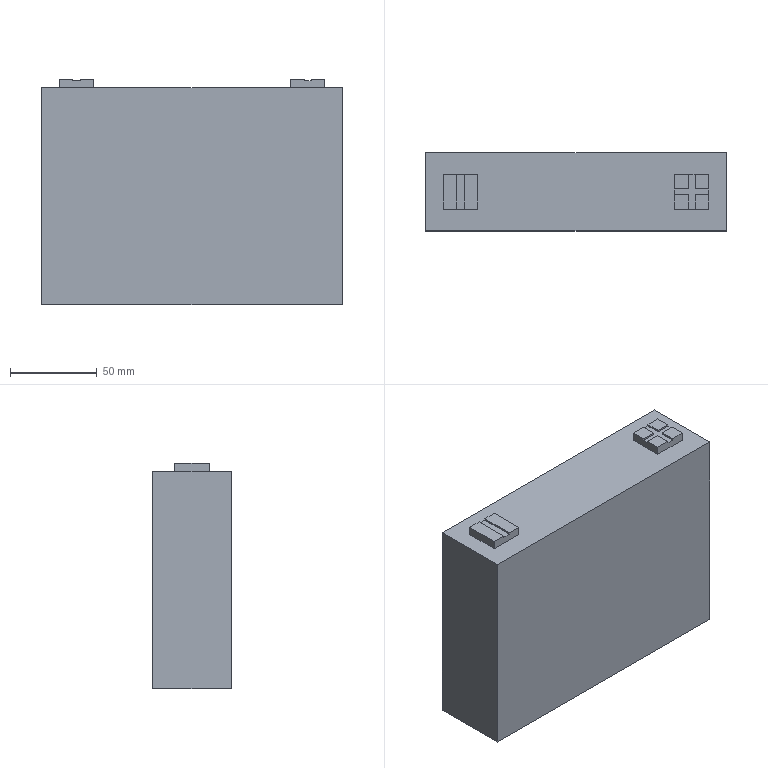Component | SolidWorks | AD12-SquareCell.SDPRT-15 | 1 solid | 32 faces | box 173 x 45 x 130 mm | volume 976901 mm3 | plane 32 | material 6061-T6 (SS)
build123d program:
from build123d import *

# Parameters (mm, degrees)
SKETCH1_W           = 173
SKETCH1_H           = 45
BOSS_EXTRUDE1_DEPTH = 125
SKETCH2_W           = 20
SKETCH2_H           = 20
BOSS_EXTRUDE2_DEPTH = 5
SKETCH3_W           = 4.63
SKETCH3_H           = 20
CUT_EXTRUDE1_DEPTH  = 1


with BuildPart() as part:
    # Sketch1 → Boss-Extrude1 (new body)
    with BuildSketch(Plane.XY):
        with Locations((86.5, 22.5)):
            Rectangle(SKETCH1_W, SKETCH1_H)
    extrude(amount=BOSS_EXTRUDE1_DEPTH)

    # Sketch2 → Boss-Extrude2 (add)
    with BuildSketch(Plane.XY.offset(125)):
        with Locations((153, 22.5)):
            Rectangle(SKETCH2_W, SKETCH2_H)
        with Locations((20, 22.5)):
            Rectangle(SKETCH2_W, SKETCH2_H)
    extrude(amount=BOSS_EXTRUDE2_DEPTH)

    # Sketch3 → Cut-Extrude1 (cut)
    with BuildSketch(Plane.XY.offset(130)):
        Polygon((143, 24.199), (151.25, 24.199), (151.25, 32.5), (155.042, 32.5), (155.042, 24.199), (163, 24.199), (163, 20.751), (155.042, 20.751), (155.042, 12.5), (151.25, 12.5), (151.25, 20.751), (143, 20.751), align=None)
        with Locations((19.957, 22.5)):
            Rectangle(SKETCH3_W, SKETCH3_H)
    extrude(amount=-CUT_EXTRUDE1_DEPTH, mode=Mode.SUBTRACT)


solid = part.part

# Placed as in the assembly
solid = solid.moved(Location((-374.414, -123.961, 199.12), (0, 0, 0)))
STEP:
#1=COLOUR_RGB('',0.7922,0.8196,0.9333);
#2=FILL_AREA_STYLE_COLOUR('',#1);
#3=FILL_AREA_STYLE('',(#2));
#4=SURFACE_STYLE_FILL_AREA(#3);
#5=SURFACE_SIDE_STYLE('',(#4));
#6=SURFACE_STYLE_USAGE(.BOTH.,#5);
#7=PRESENTATION_STYLE_ASSIGNMENT((#6));
#8=CARTESIAN_POINT('',(-14.046,-3.601,12.957));
#9=VERTEX_POINT('',#8);
#10=CARTESIAN_POINT('',(-14.046,-4.388,12.957));
#11=VERTEX_POINT('',#10);
#12=CARTESIAN_POINT('',(-14.046,-3.601,12.957));
#13=DIRECTION('',(0.,-1.,0.));
#14=VECTOR('',#13,39.37);
#15=LINE('',#12,#14);
#16=EDGE_CURVE('',#9,#11,#15,.T.);
#17=ORIENTED_EDGE('',*,*,#16,.F.);
#18=CARTESIAN_POINT('',(-14.347,-3.601,12.957));
#19=VERTEX_POINT('',#18);
#20=CARTESIAN_POINT('',(-14.347,-3.601,12.957));
#21=DIRECTION('',(-1.,0.,0.));
#22=VECTOR('',#21,39.37);
#23=LINE('',#20,#22);
#24=EDGE_CURVE('',#9,#19,#23,.T.);
#25=ORIENTED_EDGE('',*,*,#24,.T.);
#26=CARTESIAN_POINT('',(-14.347,-4.388,12.957));
#27=VERTEX_POINT('',#26);
#28=CARTESIAN_POINT('',(-14.347,-3.601,12.957));
#29=DIRECTION('',(0.,-1.,0.));
#30=VECTOR('',#29,39.37);
#31=LINE('',#28,#30);
#32=EDGE_CURVE('',#19,#27,#31,.T.);
#33=ORIENTED_EDGE('',*,*,#32,.T.);
#34=CARTESIAN_POINT('',(-14.347,-4.388,12.957));
#35=DIRECTION('',(1.,0.,0.));
#36=VECTOR('',#35,39.37);
#37=LINE('',#34,#36);
#38=EDGE_CURVE('',#27,#11,#37,.T.);
#39=ORIENTED_EDGE('',*,*,#38,.T.);
#40=EDGE_LOOP('',(#17,#25,#33,#39));
#41=FACE_OUTER_BOUND('',#40,.T.);
#42=CARTESIAN_POINT('',(-14.741,-4.88,12.957));
#43=DIRECTION('',(0.,0.,1.));
#44=DIRECTION('',(1.,0.,0.));
#45=AXIS2_PLACEMENT_3D('',#42,#43,#44);
#46=PLANE('',#45);
#47=ADVANCED_FACE('',(#41),#46,.T.);
#48=CARTESIAN_POINT('',(-8.786,-3.928,12.957));
#49=VERTEX_POINT('',#48);
#50=CARTESIAN_POINT('',(-9.111,-3.928,12.957));
#51=VERTEX_POINT('',#50);
#52=CARTESIAN_POINT('',(-9.111,-3.928,12.957));
#53=DIRECTION('',(-1.,0.,0.));
#54=VECTOR('',#53,39.37);
#55=LINE('',#52,#54);
#56=EDGE_CURVE('',#49,#51,#55,.T.);
#57=ORIENTED_EDGE('',*,*,#56,.F.);
#58=CARTESIAN_POINT('',(-8.786,-3.601,12.957));
#59=VERTEX_POINT('',#58);
#60=CARTESIAN_POINT('',(-8.786,-3.601,12.957));
#61=DIRECTION('',(0.,-1.,0.));
#62=VECTOR('',#61,39.37);
#63=LINE('',#60,#62);
#64=EDGE_CURVE('',#59,#49,#63,.T.);
#65=ORIENTED_EDGE('',*,*,#64,.F.);
#66=CARTESIAN_POINT('',(-9.111,-3.601,12.957));
#67=VERTEX_POINT('',#66);
#68=CARTESIAN_POINT('',(-9.111,-3.601,12.957));
#69=DIRECTION('',(-1.,0.,0.));
#70=VECTOR('',#69,39.37);
#71=LINE('',#68,#70);
#72=EDGE_CURVE('',#59,#67,#71,.T.);
#73=ORIENTED_EDGE('',*,*,#72,.T.);
#74=CARTESIAN_POINT('',(-9.111,-3.601,12.957));
#75=DIRECTION('',(0.,-1.,0.));
#76=VECTOR('',#75,39.37);
#77=LINE('',#74,#76);
#78=EDGE_CURVE('',#67,#51,#77,.T.);
#79=ORIENTED_EDGE('',*,*,#78,.T.);
#80=EDGE_LOOP('',(#57,#65,#73,#79));
#81=FACE_OUTER_BOUND('',#80,.T.);
#82=CARTESIAN_POINT('',(-14.741,-4.88,12.957));
#83=DIRECTION('',(0.,0.,1.));
#84=DIRECTION('',(1.,0.,0.));
#85=AXIS2_PLACEMENT_3D('',#82,#83,#84);
#86=PLANE('',#85);
#87=ADVANCED_FACE('',(#81),#86,.T.);
#88=CARTESIAN_POINT('',(-8.637,-3.928,12.957));
#89=VERTEX_POINT('',#88);
#90=CARTESIAN_POINT('',(-8.637,-3.601,12.957));
#91=VERTEX_POINT('',#90);
#92=CARTESIAN_POINT('',(-8.637,-3.601,12.957));
#93=DIRECTION('',(0.,1.,0.));
#94=VECTOR('',#93,39.37);
#95=LINE('',#92,#94);
#96=EDGE_CURVE('',#89,#91,#95,.T.);
#97=ORIENTED_EDGE('',*,*,#96,.F.);
#98=CARTESIAN_POINT('',(-8.323,-3.928,12.957));
#99=VERTEX_POINT('',#98);
#100=CARTESIAN_POINT('',(-8.637,-3.928,12.957));
#101=DIRECTION('',(-1.,0.,0.));
#102=VECTOR('',#101,39.37);
#103=LINE('',#100,#102);
#104=EDGE_CURVE('',#99,#89,#103,.T.);
#105=ORIENTED_EDGE('',*,*,#104,.F.);
#106=CARTESIAN_POINT('',(-8.323,-3.601,12.957));
#107=VERTEX_POINT('',#106);
#108=CARTESIAN_POINT('',(-8.323,-3.601,12.957));
#109=DIRECTION('',(0.,1.,0.));
#110=VECTOR('',#109,39.37);
#111=LINE('',#108,#110);
#112=EDGE_CURVE('',#99,#107,#111,.T.);
#113=ORIENTED_EDGE('',*,*,#112,.T.);
#114=CARTESIAN_POINT('',(-9.111,-3.601,12.957));
#115=DIRECTION('',(-1.,0.,0.));
#116=VECTOR('',#115,39.37);
#117=LINE('',#114,#116);
#118=EDGE_CURVE('',#107,#91,#117,.T.);
#119=ORIENTED_EDGE('',*,*,#118,.T.);
#120=EDGE_LOOP('',(#97,#105,#113,#119));
#121=FACE_OUTER_BOUND('',#120,.T.);
#122=CARTESIAN_POINT('',(-14.741,-4.88,12.957));
#123=DIRECTION('',(0.,0.,1.));
#124=DIRECTION('',(1.,0.,0.));
#125=AXIS2_PLACEMENT_3D('',#122,#123,#124);
#126=PLANE('',#125);
#127=ADVANCED_FACE('',(#121),#126,.T.);
#128=CARTESIAN_POINT('',(-8.637,-4.063,12.957));
#129=VERTEX_POINT('',#128);
#130=CARTESIAN_POINT('',(-8.323,-4.063,12.957));
#131=VERTEX_POINT('',#130);
#132=CARTESIAN_POINT('',(-8.637,-4.063,12.957));
#133=DIRECTION('',(1.,0.,0.));
#134=VECTOR('',#133,39.37);
#135=LINE('',#132,#134);
#136=EDGE_CURVE('',#129,#131,#135,.T.);
#137=ORIENTED_EDGE('',*,*,#136,.F.);
#138=CARTESIAN_POINT('',(-8.637,-4.388,12.957));
#139=VERTEX_POINT('',#138);
#140=CARTESIAN_POINT('',(-8.637,-4.063,12.957));
#141=DIRECTION('',(0.,1.,0.));
#142=VECTOR('',#141,39.37);
#143=LINE('',#140,#142);
#144=EDGE_CURVE('',#139,#129,#143,.T.);
#145=ORIENTED_EDGE('',*,*,#144,.F.);
#146=CARTESIAN_POINT('',(-8.323,-4.388,12.957));
#147=VERTEX_POINT('',#146);
#148=CARTESIAN_POINT('',(-9.111,-4.388,12.957));
#149=DIRECTION('',(1.,0.,0.));
#150=VECTOR('',#149,39.37);
#151=LINE('',#148,#150);
#152=EDGE_CURVE('',#139,#147,#151,.T.);
#153=ORIENTED_EDGE('',*,*,#152,.T.);
#154=CARTESIAN_POINT('',(-8.323,-3.601,12.957));
#155=DIRECTION('',(0.,1.,0.));
#156=VECTOR('',#155,39.37);
#157=LINE('',#154,#156);
#158=EDGE_CURVE('',#147,#131,#157,.T.);
#159=ORIENTED_EDGE('',*,*,#158,.T.);
#160=EDGE_LOOP('',(#137,#145,#153,#159));
#161=FACE_OUTER_BOUND('',#160,.T.);
#162=CARTESIAN_POINT('',(-14.741,-4.88,12.957));
#163=DIRECTION('',(0.,0.,1.));
#164=DIRECTION('',(1.,0.,0.));
#165=AXIS2_PLACEMENT_3D('',#162,#163,#164);
#166=PLANE('',#165);
#167=ADVANCED_FACE('',(#161),#166,.T.);
#168=CARTESIAN_POINT('',(-9.111,-3.601,12.761));
#169=VERTEX_POINT('',#168);
#170=CARTESIAN_POINT('',(-9.111,-4.388,12.761));
#171=VERTEX_POINT('',#170);
#172=CARTESIAN_POINT('',(-9.111,-3.601,12.761));
#173=DIRECTION('',(0.,-1.,0.));
#174=VECTOR('',#173,39.37);
#175=LINE('',#172,#174);
#176=EDGE_CURVE('',#169,#171,#175,.T.);
#177=ORIENTED_EDGE('',*,*,#176,.F.);
#178=CARTESIAN_POINT('',(-8.323,-3.601,12.761));
#179=VERTEX_POINT('',#178);
#180=CARTESIAN_POINT('',(-9.111,-3.601,12.761));
#181=DIRECTION('',(-1.,0.,0.));
#182=VECTOR('',#181,39.37);
#183=LINE('',#180,#182);
#184=EDGE_CURVE('',#179,#169,#183,.T.);
#185=ORIENTED_EDGE('',*,*,#184,.F.);
#186=CARTESIAN_POINT('',(-8.323,-4.388,12.761));
#187=VERTEX_POINT('',#186);
#188=CARTESIAN_POINT('',(-8.323,-3.601,12.761));
#189=DIRECTION('',(0.,1.,0.));
#190=VECTOR('',#189,39.37);
#191=LINE('',#188,#190);
#192=EDGE_CURVE('',#187,#179,#191,.T.);
#193=ORIENTED_EDGE('',*,*,#192,.F.);
#194=CARTESIAN_POINT('',(-9.111,-4.388,12.761));
#195=DIRECTION('',(1.,0.,0.));
#196=VECTOR('',#195,39.37);
#197=LINE('',#194,#196);
#198=EDGE_CURVE('',#171,#187,#197,.T.);
#199=ORIENTED_EDGE('',*,*,#198,.F.);
#200=EDGE_LOOP('',(#177,#185,#193,#199));
#201=FACE_BOUND('',#200,.T.);
#202=CARTESIAN_POINT('',(-14.741,-3.109,12.761));
#203=VERTEX_POINT('',#202);
#204=CARTESIAN_POINT('',(-14.741,-4.88,12.761));
#205=VERTEX_POINT('',#204);
#206=CARTESIAN_POINT('',(-14.741,-4.88,12.761));
#207=DIRECTION('',(-0.,-1.,0.));
#208=VECTOR('',#207,39.37);
#209=LINE('',#206,#208);
#210=EDGE_CURVE('',#203,#205,#209,.T.);
#211=ORIENTED_EDGE('',*,*,#210,.T.);
#212=CARTESIAN_POINT('',(-7.93,-4.88,12.761));
#213=VERTEX_POINT('',#212);
#214=CARTESIAN_POINT('',(-14.741,-4.88,12.761));
#215=DIRECTION('',(1.,0.,0.));
#216=VECTOR('',#215,39.37);
#217=LINE('',#214,#216);
#218=EDGE_CURVE('',#205,#213,#217,.T.);
#219=ORIENTED_EDGE('',*,*,#218,.T.);
#220=CARTESIAN_POINT('',(-7.93,-3.109,12.761));
#221=VERTEX_POINT('',#220);
#222=CARTESIAN_POINT('',(-7.93,-4.88,12.761));
#223=DIRECTION('',(0.,1.,0.));
#224=VECTOR('',#223,39.37);
#225=LINE('',#222,#224);
#226=EDGE_CURVE('',#213,#221,#225,.T.);
#227=ORIENTED_EDGE('',*,*,#226,.T.);
#228=CARTESIAN_POINT('',(-14.741,-3.109,12.761));
#229=DIRECTION('',(-1.,0.,0.));
#230=VECTOR('',#229,39.37);
#231=LINE('',#228,#230);
#232=EDGE_CURVE('',#221,#203,#231,.T.);
#233=ORIENTED_EDGE('',*,*,#232,.T.);
#234=EDGE_LOOP('',(#211,#219,#227,#233));
#235=FACE_OUTER_BOUND('',#234,.T.);
#236=CARTESIAN_POINT('',(-14.347,-3.601,12.761));
#237=VERTEX_POINT('',#236);
#238=CARTESIAN_POINT('',(-14.347,-4.388,12.761));
#239=VERTEX_POINT('',#238);
#240=CARTESIAN_POINT('',(-14.347,-3.601,12.761));
#241=DIRECTION('',(0.,-1.,0.));
#242=VECTOR('',#241,39.37);
#243=LINE('',#240,#242);
#244=EDGE_CURVE('',#237,#239,#243,.T.);
#245=ORIENTED_EDGE('',*,*,#244,.F.);
#246=CARTESIAN_POINT('',(-13.56,-3.601,12.761));
#247=VERTEX_POINT('',#246);
#248=CARTESIAN_POINT('',(-14.347,-3.601,12.761));
#249=DIRECTION('',(-1.,0.,0.));
#250=VECTOR('',#249,39.37);
#251=LINE('',#248,#250);
#252=EDGE_CURVE('',#247,#237,#251,.T.);
#253=ORIENTED_EDGE('',*,*,#252,.F.);
#254=CARTESIAN_POINT('',(-13.56,-4.388,12.761));
#255=VERTEX_POINT('',#254);
#256=CARTESIAN_POINT('',(-13.56,-3.601,12.761));
#257=DIRECTION('',(-0.,1.,0.));
#258=VECTOR('',#257,39.37);
#259=LINE('',#256,#258);
#260=EDGE_CURVE('',#255,#247,#259,.T.);
#261=ORIENTED_EDGE('',*,*,#260,.F.);
#262=CARTESIAN_POINT('',(-14.347,-4.388,12.761));
#263=DIRECTION('',(1.,0.,0.));
#264=VECTOR('',#263,39.37);
#265=LINE('',#262,#264);
#266=EDGE_CURVE('',#239,#255,#265,.T.);
#267=ORIENTED_EDGE('',*,*,#266,.F.);
#268=EDGE_LOOP('',(#245,#253,#261,#267));
#269=FACE_BOUND('',#268,.T.);
#270=CARTESIAN_POINT('',(-14.741,-4.88,12.761));
#271=DIRECTION('',(0.,0.,-1.));
#272=DIRECTION('',(-1.,0.,0.));
#273=AXIS2_PLACEMENT_3D('',#270,#271,#272);
#274=PLANE('',#273);
#275=ADVANCED_FACE('',(#201,#235,#269),#274,.F.);
#276=CARTESIAN_POINT('',(-14.741,-3.109,7.839));
#277=VERTEX_POINT('',#276);
#278=CARTESIAN_POINT('',(-14.741,-4.88,7.839));
#279=VERTEX_POINT('',#278);
#280=CARTESIAN_POINT('',(-14.741,-4.88,7.839));
#281=DIRECTION('',(-0.,-1.,0.));
#282=VECTOR('',#281,39.37);
#283=LINE('',#280,#282);
#284=EDGE_CURVE('',#277,#279,#283,.T.);
#285=ORIENTED_EDGE('',*,*,#284,.T.);
#286=CARTESIAN_POINT('',(-14.741,-4.88,12.761));
#287=DIRECTION('',(0.,0.,-1.));
#288=VECTOR('',#287,39.37);
#289=LINE('',#286,#288);
#290=EDGE_CURVE('',#205,#279,#289,.T.);
#291=ORIENTED_EDGE('',*,*,#290,.F.);
#292=ORIENTED_EDGE('',*,*,#210,.F.);
#293=CARTESIAN_POINT('',(-14.741,-3.109,12.761));
#294=DIRECTION('',(0.,0.,-1.));
#295=VECTOR('',#294,39.37);
#296=LINE('',#293,#295);
#297=EDGE_CURVE('',#203,#277,#296,.T.);
#298=ORIENTED_EDGE('',*,*,#297,.T.);
#299=EDGE_LOOP('',(#285,#291,#292,#298));
#300=FACE_OUTER_BOUND('',#299,.T.);
#301=CARTESIAN_POINT('',(-14.741,-4.88,12.761));
#302=DIRECTION('',(1.,-0.,0.));
#303=DIRECTION('',(0.,1.,0.));
#304=AXIS2_PLACEMENT_3D('',#301,#302,#303);
#305=PLANE('',#304);
#306=ADVANCED_FACE('',(#300),#305,.F.);
#307=CARTESIAN_POINT('',(-7.93,-4.88,7.839));
#308=VERTEX_POINT('',#307);
#309=CARTESIAN_POINT('',(-14.741,-4.88,7.839));
#310=DIRECTION('',(1.,0.,0.));
#311=VECTOR('',#310,39.37);
#312=LINE('',#309,#311);
#313=EDGE_CURVE('',#279,#308,#312,.T.);
#314=ORIENTED_EDGE('',*,*,#313,.T.);
#315=CARTESIAN_POINT('',(-7.93,-4.88,12.761));
#316=DIRECTION('',(0.,0.,-1.));
#317=VECTOR('',#316,39.37);
#318=LINE('',#315,#317);
#319=EDGE_CURVE('',#213,#308,#318,.T.);
#320=ORIENTED_EDGE('',*,*,#319,.F.);
#321=ORIENTED_EDGE('',*,*,#218,.F.);
#322=ORIENTED_EDGE('',*,*,#290,.T.);
#323=EDGE_LOOP('',(#314,#320,#321,#322));
#324=FACE_OUTER_BOUND('',#323,.T.);
#325=CARTESIAN_POINT('',(-14.741,-4.88,12.761));
#326=DIRECTION('',(0.,1.,0.));
#327=DIRECTION('',(0.,0.,1.));
#328=AXIS2_PLACEMENT_3D('',#325,#326,#327);
#329=PLANE('',#328);
#330=ADVANCED_FACE('',(#324),#329,.F.);
#331=CARTESIAN_POINT('',(-7.93,-3.109,7.839));
#332=VERTEX_POINT('',#331);
#333=CARTESIAN_POINT('',(-7.93,-4.88,7.839));
#334=DIRECTION('',(0.,1.,0.));
#335=VECTOR('',#334,39.37);
#336=LINE('',#333,#335);
#337=EDGE_CURVE('',#308,#332,#336,.T.);
#338=ORIENTED_EDGE('',*,*,#337,.T.);
#339=CARTESIAN_POINT('',(-7.93,-3.109,12.761));
#340=DIRECTION('',(0.,0.,-1.));
#341=VECTOR('',#340,39.37);
#342=LINE('',#339,#341);
#343=EDGE_CURVE('',#221,#332,#342,.T.);
#344=ORIENTED_EDGE('',*,*,#343,.F.);
#345=ORIENTED_EDGE('',*,*,#226,.F.);
#346=ORIENTED_EDGE('',*,*,#319,.T.);
#347=EDGE_LOOP('',(#338,#344,#345,#346));
#348=FACE_OUTER_BOUND('',#347,.T.);
#349=CARTESIAN_POINT('',(-7.93,-4.88,12.761));
#350=DIRECTION('',(-1.,0.,0.));
#351=DIRECTION('',(-0.,-1.,0.));
#352=AXIS2_PLACEMENT_3D('',#349,#350,#351);
#353=PLANE('',#352);
#354=ADVANCED_FACE('',(#348),#353,.F.);
#355=CARTESIAN_POINT('',(-14.741,-3.109,7.839));
#356=DIRECTION('',(-1.,0.,0.));
#357=VECTOR('',#356,39.37);
#358=LINE('',#355,#357);
#359=EDGE_CURVE('',#332,#277,#358,.T.);
#360=ORIENTED_EDGE('',*,*,#359,.T.);
#361=ORIENTED_EDGE('',*,*,#297,.F.);
#362=ORIENTED_EDGE('',*,*,#232,.F.);
#363=ORIENTED_EDGE('',*,*,#343,.T.);
#364=EDGE_LOOP('',(#360,#361,#362,#363));
#365=FACE_OUTER_BOUND('',#364,.T.);
#366=CARTESIAN_POINT('',(-14.741,-3.109,12.761));
#367=DIRECTION('',(0.,-1.,0.));
#368=DIRECTION('',(0.,0.,-1.));
#369=AXIS2_PLACEMENT_3D('',#366,#367,#368);
#370=PLANE('',#369);
#371=ADVANCED_FACE('',(#365),#370,.F.);
#372=ORIENTED_EDGE('',*,*,#284,.F.);
#373=ORIENTED_EDGE('',*,*,#359,.F.);
#374=ORIENTED_EDGE('',*,*,#337,.F.);
#375=ORIENTED_EDGE('',*,*,#313,.F.);
#376=EDGE_LOOP('',(#372,#373,#374,#375));
#377=FACE_OUTER_BOUND('',#376,.T.);
#378=CARTESIAN_POINT('',(-14.741,-4.88,7.839));
#379=DIRECTION('',(0.,0.,-1.));
#380=DIRECTION('',(-1.,0.,0.));
#381=AXIS2_PLACEMENT_3D('',#378,#379,#380);
#382=PLANE('',#381);
#383=ADVANCED_FACE('',(#377),#382,.T.);
#384=CARTESIAN_POINT('',(-9.111,-3.928,12.918));
#385=VERTEX_POINT('',#384);
#386=CARTESIAN_POINT('',(-9.111,-4.063,12.918));
#387=VERTEX_POINT('',#386);
#388=CARTESIAN_POINT('',(-9.111,-3.928,12.918));
#389=DIRECTION('',(0.,-1.,0.));
#390=VECTOR('',#389,39.37);
#391=LINE('',#388,#390);
#392=EDGE_CURVE('',#385,#387,#391,.T.);
#393=ORIENTED_EDGE('',*,*,#392,.F.);
#394=CARTESIAN_POINT('',(-9.111,-3.928,12.918));
#395=DIRECTION('',(0.,0.,1.));
#396=VECTOR('',#395,39.37);
#397=LINE('',#394,#396);
#398=EDGE_CURVE('',#385,#51,#397,.T.);
#399=ORIENTED_EDGE('',*,*,#398,.T.);
#400=ORIENTED_EDGE('',*,*,#78,.F.);
#401=CARTESIAN_POINT('',(-9.111,-3.601,12.957));
#402=DIRECTION('',(0.,0.,-1.));
#403=VECTOR('',#402,39.37);
#404=LINE('',#401,#403);
#405=EDGE_CURVE('',#67,#169,#404,.T.);
#406=ORIENTED_EDGE('',*,*,#405,.T.);
#407=ORIENTED_EDGE('',*,*,#176,.T.);
#408=CARTESIAN_POINT('',(-9.111,-4.388,12.957));
#409=VERTEX_POINT('',#408);
#410=CARTESIAN_POINT('',(-9.111,-4.388,12.957));
#411=DIRECTION('',(0.,0.,-1.));
#412=VECTOR('',#411,39.37);
#413=LINE('',#410,#412);
#414=EDGE_CURVE('',#409,#171,#413,.T.);
#415=ORIENTED_EDGE('',*,*,#414,.F.);
#416=CARTESIAN_POINT('',(-9.111,-4.063,12.957));
#417=VERTEX_POINT('',#416);
#418=CARTESIAN_POINT('',(-9.111,-3.601,12.957));
#419=DIRECTION('',(0.,-1.,0.));
#420=VECTOR('',#419,39.37);
#421=LINE('',#418,#420);
#422=EDGE_CURVE('',#417,#409,#421,.T.);
#423=ORIENTED_EDGE('',*,*,#422,.F.);
#424=CARTESIAN_POINT('',(-9.111,-4.063,12.918));
#425=DIRECTION('',(0.,0.,1.));
#426=VECTOR('',#425,39.37);
#427=LINE('',#424,#426);
#428=EDGE_CURVE('',#387,#417,#427,.T.);
#429=ORIENTED_EDGE('',*,*,#428,.F.);
#430=EDGE_LOOP('',(#393,#399,#400,#406,#407,#415,#423,#429));
#431=FACE_OUTER_BOUND('',#430,.T.);
#432=CARTESIAN_POINT('',(-9.111,-3.601,12.957));
#433=DIRECTION('',(1.,0.,0.));
#434=DIRECTION('',(0.,0.,-1.));
#435=AXIS2_PLACEMENT_3D('',#432,#433,#434);
#436=PLANE('',#435);
#437=ADVANCED_FACE('',(#431),#436,.F.);
#438=ORIENTED_EDGE('',*,*,#152,.F.);
#439=CARTESIAN_POINT('',(-8.637,-4.388,12.918));
#440=VERTEX_POINT('',#439);
#441=CARTESIAN_POINT('',(-8.637,-4.388,12.918));
#442=DIRECTION('',(0.,0.,1.));
#443=VECTOR('',#442,39.37);
#444=LINE('',#441,#443);
#445=EDGE_CURVE('',#440,#139,#444,.T.);
#446=ORIENTED_EDGE('',*,*,#445,.F.);
#447=CARTESIAN_POINT('',(-8.786,-4.388,12.918));
#448=VERTEX_POINT('',#447);
#449=CARTESIAN_POINT('',(-8.786,-4.388,12.918));
#450=DIRECTION('',(1.,0.,0.));
#451=VECTOR('',#450,39.37);
#452=LINE('',#449,#451);
#453=EDGE_CURVE('',#448,#440,#452,.T.);
#454=ORIENTED_EDGE('',*,*,#453,.F.);
#455=CARTESIAN_POINT('',(-8.786,-4.388,12.957));
#456=VERTEX_POINT('',#455);
#457=CARTESIAN_POINT('',(-8.786,-4.388,12.918));
#458=DIRECTION('',(0.,0.,1.));
#459=VECTOR('',#458,39.37);
#460=LINE('',#457,#459);
#461=EDGE_CURVE('',#448,#456,#460,.T.);
#462=ORIENTED_EDGE('',*,*,#461,.T.);
#463=CARTESIAN_POINT('',(-9.111,-4.388,12.957));
#464=DIRECTION('',(1.,0.,0.));
#465=VECTOR('',#464,39.37);
#466=LINE('',#463,#465);
#467=EDGE_CURVE('',#409,#456,#466,.T.);
#468=ORIENTED_EDGE('',*,*,#467,.F.);
#469=ORIENTED_EDGE('',*,*,#414,.T.);
#470=ORIENTED_EDGE('',*,*,#198,.T.);
#471=CARTESIAN_POINT('',(-8.323,-4.388,12.957));
#472=DIRECTION('',(0.,0.,-1.));
#473=VECTOR('',#472,39.37);
#474=LINE('',#471,#473);
#475=EDGE_CURVE('',#147,#187,#474,.T.);
#476=ORIENTED_EDGE('',*,*,#475,.F.);
#477=EDGE_LOOP('',(#438,#446,#454,#462,#468,#469,#470,#476));
#478=FACE_OUTER_BOUND('',#477,.T.);
#479=CARTESIAN_POINT('',(-9.111,-4.388,12.957));
#480=DIRECTION('',(0.,1.,0.));
#481=DIRECTION('',(0.,0.,1.));
#482=AXIS2_PLACEMENT_3D('',#479,#480,#481);
#483=PLANE('',#482);
#484=ADVANCED_FACE('',(#478),#483,.F.);
#485=ORIENTED_EDGE('',*,*,#112,.F.);
#486=CARTESIAN_POINT('',(-8.323,-3.928,12.918));
#487=VERTEX_POINT('',#486);
#488=CARTESIAN_POINT('',(-8.323,-3.928,12.918));
#489=DIRECTION('',(0.,0.,1.));
#490=VECTOR('',#489,39.37);
#491=LINE('',#488,#490);
#492=EDGE_CURVE('',#487,#99,#491,.T.);
#493=ORIENTED_EDGE('',*,*,#492,.F.);
#494=CARTESIAN_POINT('',(-8.323,-4.063,12.918));
#495=VERTEX_POINT('',#494);
#496=CARTESIAN_POINT('',(-8.323,-3.928,12.918));
#497=DIRECTION('',(0.,1.,0.));
#498=VECTOR('',#497,39.37);
#499=LINE('',#496,#498);
#500=EDGE_CURVE('',#495,#487,#499,.T.);
#501=ORIENTED_EDGE('',*,*,#500,.F.);
#502=CARTESIAN_POINT('',(-8.323,-4.063,12.918));
#503=DIRECTION('',(0.,0.,1.));
#504=VECTOR('',#503,39.37);
#505=LINE('',#502,#504);
#506=EDGE_CURVE('',#495,#131,#505,.T.);
#507=ORIENTED_EDGE('',*,*,#506,.T.);
#508=ORIENTED_EDGE('',*,*,#158,.F.);
#509=ORIENTED_EDGE('',*,*,#475,.T.);
#510=ORIENTED_EDGE('',*,*,#192,.T.);
#511=CARTESIAN_POINT('',(-8.323,-3.601,12.957));
#512=DIRECTION('',(0.,0.,-1.));
#513=VECTOR('',#512,39.37);
#514=LINE('',#511,#513);
#515=EDGE_CURVE('',#107,#179,#514,.T.);
#516=ORIENTED_EDGE('',*,*,#515,.F.);
#517=EDGE_LOOP('',(#485,#493,#501,#507,#508,#509,#510,#516));
#518=FACE_OUTER_BOUND('',#517,.T.);
#519=CARTESIAN_POINT('',(-8.323,-3.601,12.957));
#520=DIRECTION('',(-1.,0.,0.));
#521=DIRECTION('',(0.,0.,1.));
#522=AXIS2_PLACEMENT_3D('',#519,#520,#521);
#523=PLANE('',#522);
#524=ADVANCED_FACE('',(#518),#523,.F.);
#525=ORIENTED_EDGE('',*,*,#72,.F.);
#526=CARTESIAN_POINT('',(-8.786,-3.601,12.918));
#527=VERTEX_POINT('',#526);
#528=CARTESIAN_POINT('',(-8.786,-3.601,12.918));
#529=DIRECTION('',(0.,0.,1.));
#530=VECTOR('',#529,39.37);
#531=LINE('',#528,#530);
#532=EDGE_CURVE('',#527,#59,#531,.T.);
#533=ORIENTED_EDGE('',*,*,#532,.F.);
#534=CARTESIAN_POINT('',(-8.637,-3.601,12.918));
#535=VERTEX_POINT('',#534);
#536=CARTESIAN_POINT('',(-8.786,-3.601,12.918));
#537=DIRECTION('',(-1.,0.,0.));
#538=VECTOR('',#537,39.37);
#539=LINE('',#536,#538);
#540=EDGE_CURVE('',#535,#527,#539,.T.);
#541=ORIENTED_EDGE('',*,*,#540,.F.);
#542=CARTESIAN_POINT('',(-8.637,-3.601,12.918));
#543=DIRECTION('',(0.,0.,1.));
#544=VECTOR('',#543,39.37);
#545=LINE('',#542,#544);
#546=EDGE_CURVE('',#535,#91,#545,.T.);
#547=ORIENTED_EDGE('',*,*,#546,.T.);
#548=ORIENTED_EDGE('',*,*,#118,.F.);
#549=ORIENTED_EDGE('',*,*,#515,.T.);
#550=ORIENTED_EDGE('',*,*,#184,.T.);
#551=ORIENTED_EDGE('',*,*,#405,.F.);
#552=EDGE_LOOP('',(#525,#533,#541,#547,#548,#549,#550,#551));
#553=FACE_OUTER_BOUND('',#552,.T.);
#554=CARTESIAN_POINT('',(-9.111,-3.601,12.957));
#555=DIRECTION('',(0.,-1.,0.));
#556=DIRECTION('',(0.,0.,-1.));
#557=AXIS2_PLACEMENT_3D('',#554,#555,#556);
#558=PLANE('',#557);
#559=ADVANCED_FACE('',(#553),#558,.F.);
#560=CARTESIAN_POINT('',(-8.786,-4.063,12.957));
#561=VERTEX_POINT('',#560);
#562=CARTESIAN_POINT('',(-8.786,-4.063,12.957));
#563=DIRECTION('',(0.,-1.,0.));
#564=VECTOR('',#563,39.37);
#565=LINE('',#562,#564);
#566=EDGE_CURVE('',#561,#456,#565,.T.);
#567=ORIENTED_EDGE('',*,*,#566,.F.);
#568=CARTESIAN_POINT('',(-9.111,-4.063,12.957));
#569=DIRECTION('',(1.,0.,0.));
#570=VECTOR('',#569,39.37);
#571=LINE('',#568,#570);
#572=EDGE_CURVE('',#417,#561,#571,.T.);
#573=ORIENTED_EDGE('',*,*,#572,.F.);
#574=ORIENTED_EDGE('',*,*,#422,.T.);
#575=ORIENTED_EDGE('',*,*,#467,.T.);
#576=EDGE_LOOP('',(#567,#573,#574,#575));
#577=FACE_OUTER_BOUND('',#576,.T.);
#578=CARTESIAN_POINT('',(-14.741,-4.88,12.957));
#579=DIRECTION('',(0.,0.,1.));
#580=DIRECTION('',(1.,0.,0.));
#581=AXIS2_PLACEMENT_3D('',#578,#579,#580);
#582=PLANE('',#581);
#583=ADVANCED_FACE('',(#577),#582,.T.);
#584=ORIENTED_EDGE('',*,*,#244,.T.);
#585=CARTESIAN_POINT('',(-14.347,-4.388,12.957));
#586=DIRECTION('',(0.,0.,-1.));
#587=VECTOR('',#586,39.37);
#588=LINE('',#585,#587);
#589=EDGE_CURVE('',#27,#239,#588,.T.);
#590=ORIENTED_EDGE('',*,*,#589,.F.);
#591=ORIENTED_EDGE('',*,*,#32,.F.);
#592=CARTESIAN_POINT('',(-14.347,-3.601,12.957));
#593=DIRECTION('',(0.,0.,-1.));
#594=VECTOR('',#593,39.37);
#595=LINE('',#592,#594);
#596=EDGE_CURVE('',#19,#237,#595,.T.);
#597=ORIENTED_EDGE('',*,*,#596,.T.);
#598=EDGE_LOOP('',(#584,#590,#591,#597));
#599=FACE_OUTER_BOUND('',#598,.T.);
#600=CARTESIAN_POINT('',(-14.347,-3.601,12.957));
#601=DIRECTION('',(1.,0.,0.));
#602=DIRECTION('',(-0.,1.,0.));
#603=AXIS2_PLACEMENT_3D('',#600,#601,#602);
#604=PLANE('',#603);
#605=ADVANCED_FACE('',(#599),#604,.F.);
#606=CARTESIAN_POINT('',(-14.046,-4.388,12.918));
#607=VERTEX_POINT('',#606);
#608=CARTESIAN_POINT('',(-13.864,-4.388,12.918));
#609=VERTEX_POINT('',#608);
#610=CARTESIAN_POINT('',(-14.046,-4.388,12.918));
#611=DIRECTION('',(1.,0.,0.));
#612=VECTOR('',#611,39.37);
#613=LINE('',#610,#612);
#614=EDGE_CURVE('',#607,#609,#613,.T.);
#615=ORIENTED_EDGE('',*,*,#614,.F.);
#616=CARTESIAN_POINT('',(-14.046,-4.388,12.918));
#617=DIRECTION('',(0.,0.,1.));
#618=VECTOR('',#617,39.37);
#619=LINE('',#616,#618);
#620=EDGE_CURVE('',#607,#11,#619,.T.);
#621=ORIENTED_EDGE('',*,*,#620,.T.);
#622=ORIENTED_EDGE('',*,*,#38,.F.);
#623=ORIENTED_EDGE('',*,*,#589,.T.);
#624=ORIENTED_EDGE('',*,*,#266,.T.);
#625=CARTESIAN_POINT('',(-13.56,-4.388,12.957));
#626=VERTEX_POINT('',#625);
#627=CARTESIAN_POINT('',(-13.56,-4.388,12.957));
#628=DIRECTION('',(0.,0.,-1.));
#629=VECTOR('',#628,39.37);
#630=LINE('',#627,#629);
#631=EDGE_CURVE('',#626,#255,#630,.T.);
#632=ORIENTED_EDGE('',*,*,#631,.F.);
#633=CARTESIAN_POINT('',(-13.864,-4.388,12.957));
#634=VERTEX_POINT('',#633);
#635=CARTESIAN_POINT('',(-14.347,-4.388,12.957));
#636=DIRECTION('',(1.,0.,0.));
#637=VECTOR('',#636,39.37);
#638=LINE('',#635,#637);
#639=EDGE_CURVE('',#634,#626,#638,.T.);
#640=ORIENTED_EDGE('',*,*,#639,.F.);
#641=CARTESIAN_POINT('',(-13.864,-4.388,12.918));
#642=DIRECTION('',(0.,0.,1.));
#643=VECTOR('',#642,39.37);
#644=LINE('',#641,#643);
#645=EDGE_CURVE('',#609,#634,#644,.T.);
#646=ORIENTED_EDGE('',*,*,#645,.F.);
#647=EDGE_LOOP('',(#615,#621,#622,#623,#624,#632,#640,#646));
#648=FACE_OUTER_BOUND('',#647,.T.);
#649=CARTESIAN_POINT('',(-14.347,-4.388,12.957));
#650=DIRECTION('',(0.,1.,0.));
#651=DIRECTION('',(0.,0.,1.));
#652=AXIS2_PLACEMENT_3D('',#649,#650,#651);
#653=PLANE('',#652);
#654=ADVANCED_FACE('',(#648),#653,.F.);
#655=ORIENTED_EDGE('',*,*,#260,.T.);
#656=CARTESIAN_POINT('',(-13.56,-3.601,12.957));
#657=VERTEX_POINT('',#656);
#658=CARTESIAN_POINT('',(-13.56,-3.601,12.957));
#659=DIRECTION('',(0.,0.,-1.));
#660=VECTOR('',#659,39.37);
#661=LINE('',#658,#660);
#662=EDGE_CURVE('',#657,#247,#661,.T.);
#663=ORIENTED_EDGE('',*,*,#662,.F.);
#664=CARTESIAN_POINT('',(-13.56,-3.601,12.957));
#665=DIRECTION('',(-0.,1.,0.));
#666=VECTOR('',#665,39.37);
#667=LINE('',#664,#666);
#668=EDGE_CURVE('',#626,#657,#667,.T.);
#669=ORIENTED_EDGE('',*,*,#668,.F.);
#670=ORIENTED_EDGE('',*,*,#631,.T.);
#671=EDGE_LOOP('',(#655,#663,#669,#670));
#672=FACE_OUTER_BOUND('',#671,.T.);
#673=CARTESIAN_POINT('',(-13.56,-3.601,12.957));
#674=DIRECTION('',(-1.,-0.,0.));
#675=DIRECTION('',(0.,-1.,0.));
#676=AXIS2_PLACEMENT_3D('',#673,#674,#675);
#677=PLANE('',#676);
#678=ADVANCED_FACE('',(#672),#677,.F.);
#679=ORIENTED_EDGE('',*,*,#24,.F.);
#680=CARTESIAN_POINT('',(-14.046,-3.601,12.918));
#681=VERTEX_POINT('',#680);
#682=CARTESIAN_POINT('',(-14.046,-3.601,12.918));
#683=DIRECTION('',(0.,0.,1.));
#684=VECTOR('',#683,39.37);
#685=LINE('',#682,#684);
#686=EDGE_CURVE('',#681,#9,#685,.T.);
#687=ORIENTED_EDGE('',*,*,#686,.F.);
#688=CARTESIAN_POINT('',(-13.864,-3.601,12.918));
#689=VERTEX_POINT('',#688);
#690=CARTESIAN_POINT('',(-14.046,-3.601,12.918));
#691=DIRECTION('',(-1.,0.,0.));
#692=VECTOR('',#691,39.37);
#693=LINE('',#690,#692);
#694=EDGE_CURVE('',#689,#681,#693,.T.);
#695=ORIENTED_EDGE('',*,*,#694,.F.);
#696=CARTESIAN_POINT('',(-13.864,-3.601,12.957));
#697=VERTEX_POINT('',#696);
#698=CARTESIAN_POINT('',(-13.864,-3.601,12.918));
#699=DIRECTION('',(0.,0.,1.));
#700=VECTOR('',#699,39.37);
#701=LINE('',#698,#700);
#702=EDGE_CURVE('',#689,#697,#701,.T.);
#703=ORIENTED_EDGE('',*,*,#702,.T.);
#704=CARTESIAN_POINT('',(-14.347,-3.601,12.957));
#705=DIRECTION('',(-1.,0.,0.));
#706=VECTOR('',#705,39.37);
#707=LINE('',#704,#706);
#708=EDGE_CURVE('',#657,#697,#707,.T.);
#709=ORIENTED_EDGE('',*,*,#708,.F.);
#710=ORIENTED_EDGE('',*,*,#662,.T.);
#711=ORIENTED_EDGE('',*,*,#252,.T.);
#712=ORIENTED_EDGE('',*,*,#596,.F.);
#713=EDGE_LOOP('',(#679,#687,#695,#703,#709,#710,#711,#712));
#714=FACE_OUTER_BOUND('',#713,.T.);
#715=CARTESIAN_POINT('',(-14.347,-3.601,12.957));
#716=DIRECTION('',(0.,-1.,0.));
#717=DIRECTION('',(0.,0.,-1.));
#718=AXIS2_PLACEMENT_3D('',#715,#716,#717);
#719=PLANE('',#718);
#720=ADVANCED_FACE('',(#714),#719,.F.);
#721=CARTESIAN_POINT('',(-13.864,-3.601,12.957));
#722=DIRECTION('',(-0.,1.,0.));
#723=VECTOR('',#722,39.37);
#724=LINE('',#721,#723);
#725=EDGE_CURVE('',#634,#697,#724,.T.);
#726=ORIENTED_EDGE('',*,*,#725,.F.);
#727=ORIENTED_EDGE('',*,*,#639,.T.);
#728=ORIENTED_EDGE('',*,*,#668,.T.);
#729=ORIENTED_EDGE('',*,*,#708,.T.);
#730=EDGE_LOOP('',(#726,#727,#728,#729));
#731=FACE_OUTER_BOUND('',#730,.T.);
#732=CARTESIAN_POINT('',(-14.741,-4.88,12.957));
#733=DIRECTION('',(0.,0.,1.));
#734=DIRECTION('',(1.,0.,0.));
#735=AXIS2_PLACEMENT_3D('',#732,#733,#734);
#736=PLANE('',#735);
#737=ADVANCED_FACE('',(#731),#736,.T.);
#738=ORIENTED_EDGE('',*,*,#56,.T.);
#739=ORIENTED_EDGE('',*,*,#398,.F.);
#740=CARTESIAN_POINT('',(-8.786,-3.928,12.918));
#741=VERTEX_POINT('',#740);
#742=CARTESIAN_POINT('',(-9.111,-3.928,12.918));
#743=DIRECTION('',(-1.,0.,0.));
#744=VECTOR('',#743,39.37);
#745=LINE('',#742,#744);
#746=EDGE_CURVE('',#741,#385,#745,.T.);
#747=ORIENTED_EDGE('',*,*,#746,.F.);
#748=CARTESIAN_POINT('',(-8.786,-3.928,12.918));
#749=DIRECTION('',(0.,0.,1.));
#750=VECTOR('',#749,39.37);
#751=LINE('',#748,#750);
#752=EDGE_CURVE('',#741,#49,#751,.T.);
#753=ORIENTED_EDGE('',*,*,#752,.T.);
#754=EDGE_LOOP('',(#738,#739,#747,#753));
#755=FACE_OUTER_BOUND('',#754,.T.);
#756=CARTESIAN_POINT('',(-9.111,-3.928,12.918));
#757=DIRECTION('',(0.,1.,0.));
#758=DIRECTION('',(0.,0.,1.));
#759=AXIS2_PLACEMENT_3D('',#756,#757,#758);
#760=PLANE('',#759);
#761=ADVANCED_FACE('',(#755),#760,.F.);
#762=ORIENTED_EDGE('',*,*,#64,.T.);
#763=ORIENTED_EDGE('',*,*,#752,.F.);
#764=CARTESIAN_POINT('',(-8.786,-3.601,12.918));
#765=DIRECTION('',(0.,-1.,0.));
#766=VECTOR('',#765,39.37);
#767=LINE('',#764,#766);
#768=EDGE_CURVE('',#527,#741,#767,.T.);
#769=ORIENTED_EDGE('',*,*,#768,.F.);
#770=ORIENTED_EDGE('',*,*,#532,.T.);
#771=EDGE_LOOP('',(#762,#763,#769,#770));
#772=FACE_OUTER_BOUND('',#771,.T.);
#773=CARTESIAN_POINT('',(-8.786,-3.601,12.918));
#774=DIRECTION('',(-1.,0.,0.));
#775=DIRECTION('',(0.,0.,1.));
#776=AXIS2_PLACEMENT_3D('',#773,#774,#775);
#777=PLANE('',#776);
#778=ADVANCED_FACE('',(#772),#777,.F.);
#779=ORIENTED_EDGE('',*,*,#96,.T.);
#780=ORIENTED_EDGE('',*,*,#546,.F.);
#781=CARTESIAN_POINT('',(-8.637,-3.928,12.918));
#782=VERTEX_POINT('',#781);
#783=CARTESIAN_POINT('',(-8.637,-3.601,12.918));
#784=DIRECTION('',(0.,1.,0.));
#785=VECTOR('',#784,39.37);
#786=LINE('',#783,#785);
#787=EDGE_CURVE('',#782,#535,#786,.T.);
#788=ORIENTED_EDGE('',*,*,#787,.F.);
#789=CARTESIAN_POINT('',(-8.637,-3.928,12.918));
#790=DIRECTION('',(0.,0.,1.));
#791=VECTOR('',#790,39.37);
#792=LINE('',#789,#791);
#793=EDGE_CURVE('',#782,#89,#792,.T.);
#794=ORIENTED_EDGE('',*,*,#793,.T.);
#795=EDGE_LOOP('',(#779,#780,#788,#794));
#796=FACE_OUTER_BOUND('',#795,.T.);
#797=CARTESIAN_POINT('',(-8.637,-3.601,12.918));
#798=DIRECTION('',(1.,0.,0.));
#799=DIRECTION('',(0.,0.,-1.));
#800=AXIS2_PLACEMENT_3D('',#797,#798,#799);
#801=PLANE('',#800);
#802=ADVANCED_FACE('',(#796),#801,.F.);
#803=ORIENTED_EDGE('',*,*,#104,.T.);
#804=ORIENTED_EDGE('',*,*,#793,.F.);
#805=CARTESIAN_POINT('',(-8.637,-3.928,12.918));
#806=DIRECTION('',(-1.,0.,0.));
#807=VECTOR('',#806,39.37);
#808=LINE('',#805,#807);
#809=EDGE_CURVE('',#487,#782,#808,.T.);
#810=ORIENTED_EDGE('',*,*,#809,.F.);
#811=ORIENTED_EDGE('',*,*,#492,.T.);
#812=EDGE_LOOP('',(#803,#804,#810,#811));
#813=FACE_OUTER_BOUND('',#812,.T.);
#814=CARTESIAN_POINT('',(-8.637,-3.928,12.918));
#815=DIRECTION('',(0.,1.,0.));
#816=DIRECTION('',(0.,0.,1.));
#817=AXIS2_PLACEMENT_3D('',#814,#815,#816);
#818=PLANE('',#817);
#819=ADVANCED_FACE('',(#813),#818,.F.);
#820=ORIENTED_EDGE('',*,*,#136,.T.);
#821=ORIENTED_EDGE('',*,*,#506,.F.);
#822=CARTESIAN_POINT('',(-8.637,-4.063,12.918));
#823=VERTEX_POINT('',#822);
#824=CARTESIAN_POINT('',(-8.637,-4.063,12.918));
#825=DIRECTION('',(1.,0.,0.));
#826=VECTOR('',#825,39.37);
#827=LINE('',#824,#826);
#828=EDGE_CURVE('',#823,#495,#827,.T.);
#829=ORIENTED_EDGE('',*,*,#828,.F.);
#830=CARTESIAN_POINT('',(-8.637,-4.063,12.918));
#831=DIRECTION('',(0.,0.,1.));
#832=VECTOR('',#831,39.37);
#833=LINE('',#830,#832);
#834=EDGE_CURVE('',#823,#129,#833,.T.);
#835=ORIENTED_EDGE('',*,*,#834,.T.);
#836=EDGE_LOOP('',(#820,#821,#829,#835));
#837=FACE_OUTER_BOUND('',#836,.T.);
#838=CARTESIAN_POINT('',(-8.637,-4.063,12.918));
#839=DIRECTION('',(0.,-1.,0.));
#840=DIRECTION('',(0.,0.,-1.));
#841=AXIS2_PLACEMENT_3D('',#838,#839,#840);
#842=PLANE('',#841);
#843=ADVANCED_FACE('',(#837),#842,.F.);
#844=ORIENTED_EDGE('',*,*,#144,.T.);
#845=ORIENTED_EDGE('',*,*,#834,.F.);
#846=CARTESIAN_POINT('',(-8.637,-4.063,12.918));
#847=DIRECTION('',(0.,1.,0.));
#848=VECTOR('',#847,39.37);
#849=LINE('',#846,#848);
#850=EDGE_CURVE('',#440,#823,#849,.T.);
#851=ORIENTED_EDGE('',*,*,#850,.F.);
#852=ORIENTED_EDGE('',*,*,#445,.T.);
#853=EDGE_LOOP('',(#844,#845,#851,#852));
#854=FACE_OUTER_BOUND('',#853,.T.);
#855=CARTESIAN_POINT('',(-8.637,-4.063,12.918));
#856=DIRECTION('',(1.,0.,0.));
#857=DIRECTION('',(0.,0.,-1.));
#858=AXIS2_PLACEMENT_3D('',#855,#856,#857);
#859=PLANE('',#858);
#860=ADVANCED_FACE('',(#854),#859,.F.);
#861=ORIENTED_EDGE('',*,*,#566,.T.);
#862=ORIENTED_EDGE('',*,*,#461,.F.);
#863=CARTESIAN_POINT('',(-8.786,-4.063,12.918));
#864=VERTEX_POINT('',#863);
#865=CARTESIAN_POINT('',(-8.786,-4.063,12.918));
#866=DIRECTION('',(0.,-1.,0.));
#867=VECTOR('',#866,39.37);
#868=LINE('',#865,#867);
#869=EDGE_CURVE('',#864,#448,#868,.T.);
#870=ORIENTED_EDGE('',*,*,#869,.F.);
#871=CARTESIAN_POINT('',(-8.786,-4.063,12.918));
#872=DIRECTION('',(0.,0.,1.));
#873=VECTOR('',#872,39.37);
#874=LINE('',#871,#873);
#875=EDGE_CURVE('',#864,#561,#874,.T.);
#876=ORIENTED_EDGE('',*,*,#875,.T.);
#877=EDGE_LOOP('',(#861,#862,#870,#876));
#878=FACE_OUTER_BOUND('',#877,.T.);
#879=CARTESIAN_POINT('',(-8.786,-4.063,12.918));
#880=DIRECTION('',(-1.,0.,0.));
#881=DIRECTION('',(0.,0.,1.));
#882=AXIS2_PLACEMENT_3D('',#879,#880,#881);
#883=PLANE('',#882);
#884=ADVANCED_FACE('',(#878),#883,.F.);
#885=ORIENTED_EDGE('',*,*,#572,.T.);
#886=ORIENTED_EDGE('',*,*,#875,.F.);
#887=CARTESIAN_POINT('',(-9.111,-4.063,12.918));
#888=DIRECTION('',(1.,0.,0.));
#889=VECTOR('',#888,39.37);
#890=LINE('',#887,#889);
#891=EDGE_CURVE('',#387,#864,#890,.T.);
#892=ORIENTED_EDGE('',*,*,#891,.F.);
#893=ORIENTED_EDGE('',*,*,#428,.T.);
#894=EDGE_LOOP('',(#885,#886,#892,#893));
#895=FACE_OUTER_BOUND('',#894,.T.);
#896=CARTESIAN_POINT('',(-9.111,-4.063,12.918));
#897=DIRECTION('',(0.,-1.,0.));
#898=DIRECTION('',(0.,0.,-1.));
#899=AXIS2_PLACEMENT_3D('',#896,#897,#898);
#900=PLANE('',#899);
#901=ADVANCED_FACE('',(#895),#900,.F.);
#902=ORIENTED_EDGE('',*,*,#392,.T.);
#903=ORIENTED_EDGE('',*,*,#891,.T.);
#904=ORIENTED_EDGE('',*,*,#869,.T.);
#905=ORIENTED_EDGE('',*,*,#453,.T.);
#906=ORIENTED_EDGE('',*,*,#850,.T.);
#907=ORIENTED_EDGE('',*,*,#828,.T.);
#908=ORIENTED_EDGE('',*,*,#500,.T.);
#909=ORIENTED_EDGE('',*,*,#809,.T.);
#910=ORIENTED_EDGE('',*,*,#787,.T.);
#911=ORIENTED_EDGE('',*,*,#540,.T.);
#912=ORIENTED_EDGE('',*,*,#768,.T.);
#913=ORIENTED_EDGE('',*,*,#746,.T.);
#914=EDGE_LOOP('',(#902,#903,#904,#905,#906,#907,#908,#909,#910,#911,#912,#913));
#915=FACE_OUTER_BOUND('',#914,.T.);
#916=CARTESIAN_POINT('',(-14.741,-4.88,12.918));
#917=DIRECTION('',(0.,0.,1.));
#918=DIRECTION('',(1.,0.,0.));
#919=AXIS2_PLACEMENT_3D('',#916,#917,#918);
#920=PLANE('',#919);
#921=ADVANCED_FACE('',(#915),#920,.T.);
#922=ORIENTED_EDGE('',*,*,#16,.T.);
#923=ORIENTED_EDGE('',*,*,#620,.F.);
#924=CARTESIAN_POINT('',(-14.046,-3.601,12.918));
#925=DIRECTION('',(0.,-1.,0.));
#926=VECTOR('',#925,39.37);
#927=LINE('',#924,#926);
#928=EDGE_CURVE('',#681,#607,#927,.T.);
#929=ORIENTED_EDGE('',*,*,#928,.F.);
#930=ORIENTED_EDGE('',*,*,#686,.T.);
#931=EDGE_LOOP('',(#922,#923,#929,#930));
#932=FACE_OUTER_BOUND('',#931,.T.);
#933=CARTESIAN_POINT('',(-14.046,-3.601,12.918));
#934=DIRECTION('',(-1.,0.,0.));
#935=DIRECTION('',(0.,0.,1.));
#936=AXIS2_PLACEMENT_3D('',#933,#934,#935);
#937=PLANE('',#936);
#938=ADVANCED_FACE('',(#932),#937,.F.);
#939=ORIENTED_EDGE('',*,*,#725,.T.);
#940=ORIENTED_EDGE('',*,*,#702,.F.);
#941=CARTESIAN_POINT('',(-13.864,-3.601,12.918));
#942=DIRECTION('',(-0.,1.,0.));
#943=VECTOR('',#942,39.37);
#944=LINE('',#941,#943);
#945=EDGE_CURVE('',#609,#689,#944,.T.);
#946=ORIENTED_EDGE('',*,*,#945,.F.);
#947=ORIENTED_EDGE('',*,*,#645,.T.);
#948=EDGE_LOOP('',(#939,#940,#946,#947));
#949=FACE_OUTER_BOUND('',#948,.T.);
#950=CARTESIAN_POINT('',(-13.864,-3.601,12.918));
#951=DIRECTION('',(1.,0.,0.));
#952=DIRECTION('',(-0.,1.,0.));
#953=AXIS2_PLACEMENT_3D('',#950,#951,#952);
#954=PLANE('',#953);
#955=ADVANCED_FACE('',(#949),#954,.F.);
#956=ORIENTED_EDGE('',*,*,#928,.T.);
#957=ORIENTED_EDGE('',*,*,#614,.T.);
#958=ORIENTED_EDGE('',*,*,#945,.T.);
#959=ORIENTED_EDGE('',*,*,#694,.T.);
#960=EDGE_LOOP('',(#956,#957,#958,#959));
#961=FACE_OUTER_BOUND('',#960,.T.);
#962=CARTESIAN_POINT('',(-14.741,-4.88,12.918));
#963=DIRECTION('',(0.,0.,1.));
#964=DIRECTION('',(1.,0.,0.));
#965=AXIS2_PLACEMENT_3D('',#962,#963,#964);
#966=PLANE('',#965);
#967=ADVANCED_FACE('',(#961),#966,.T.);
#968=CLOSED_SHELL('',(#47,#87,#127,#167,#275,#306,#330,#354,#371,#383,#437,#484,#524,#559,#583,#605,#654,#678,#720,#737,#761,#778,#802,#819,#843,#860,#884,#901,#921,#938,#955,#967));
#969=MANIFOLD_SOLID_BREP('',#968);
#970=STYLED_ITEM('',(#7),#969);
#971=PRESENTATION_LAYER_ASSIGNMENT('','',(#970));
#972=CARTESIAN_POINT('',(0.,0.,0.));
#973=DIRECTION('',(0.,0.,1.));
#974=DIRECTION('',(1.,0.,0.));
#975=AXIS2_PLACEMENT_3D('',#972,#973,#974);
#976=(LENGTH_UNIT()NAMED_UNIT(*)SI_UNIT($,.METRE.));
#977=LENGTH_MEASURE_WITH_UNIT(LENGTH_MEASURE(0.0254),#976);
#978=DIMENSIONAL_EXPONENTS(1.,0.,0.,0.,0.,0.,0.);
#979=(CONVERSION_BASED_UNIT('',#977)LENGTH_UNIT()NAMED_UNIT(#978));
#980=UNCERTAINTY_MEASURE_WITH_UNIT(LENGTH_MEASURE(0.00001),#979,'','');
#981=(NAMED_UNIT(*)PLANE_ANGLE_UNIT()SI_UNIT($,.RADIAN.));
#982=(NAMED_UNIT(*)SI_UNIT($,.STERADIAN.)SOLID_ANGLE_UNIT());
#983=(GEOMETRIC_REPRESENTATION_CONTEXT(3)GLOBAL_UNCERTAINTY_ASSIGNED_CONTEXT((#980))GLOBAL_UNIT_ASSIGNED_CONTEXT((#979,#981,#982))REPRESENTATION_CONTEXT('',''));
#984=ADVANCED_BREP_SHAPE_REPRESENTATION('',(#969,#975),#983);
#985=(LENGTH_UNIT()NAMED_UNIT(*)SI_UNIT($,.METRE.));
#986=LENGTH_MEASURE_WITH_UNIT(LENGTH_MEASURE(0.0254),#985);
#987=DIMENSIONAL_EXPONENTS(1.,0.,0.,0.,0.,0.,0.);
#988=(CONVERSION_BASED_UNIT('',#986)LENGTH_UNIT()NAMED_UNIT(#987));
#989=UNCERTAINTY_MEASURE_WITH_UNIT(LENGTH_MEASURE(0.00001),#988,'','');
#990=(NAMED_UNIT(*)PLANE_ANGLE_UNIT()SI_UNIT($,.RADIAN.));
#991=(NAMED_UNIT(*)SI_UNIT($,.STERADIAN.)SOLID_ANGLE_UNIT());
#992=(GEOMETRIC_REPRESENTATION_CONTEXT(3)GLOBAL_UNCERTAINTY_ASSIGNED_CONTEXT((#989))GLOBAL_UNIT_ASSIGNED_CONTEXT((#988,#990,#991))REPRESENTATION_CONTEXT('',''));
#993=MECHANICAL_DESIGN_GEOMETRIC_PRESENTATION_REPRESENTATION('',(#970),#992);